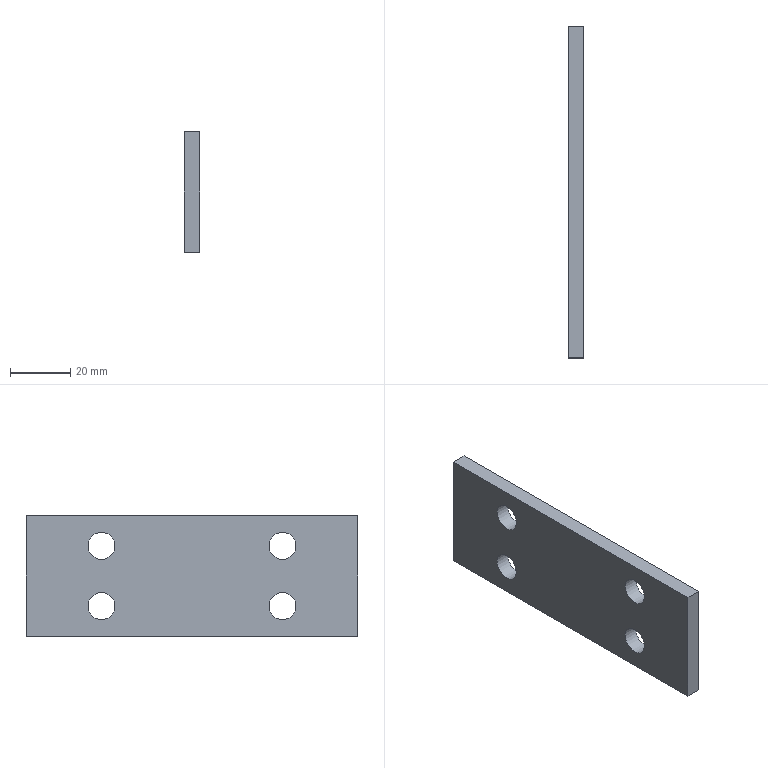Component | NX | CH3404_2-5 | 1 solid | 10 faces | box 5 x 110 x 40 mm | volume 20728 mm3 | plane 6 | cylinder 4 | commonest cylinder face diameters 9 x4
STEP:
#1=CARTESIAN_POINT('',(0.,0.,0.));
#2=DIRECTION('',(0.,0.,1.));
#3=DIRECTION('',(1.,0.,0.));
#4=AXIS2_PLACEMENT_3D('',#1,#2,#3);
#5=CARTESIAN_POINT('',(58.,-55.,20.));
#6=VERTEX_POINT('',#5);
#7=CARTESIAN_POINT('',(58.,-55.,-20.));
#8=VERTEX_POINT('',#7);
#9=CARTESIAN_POINT('',(58.,-55.,20.));
#10=DIRECTION('',(0.,0.,-1.));
#11=VECTOR('',#10,1.);
#12=LINE('',#9,#11);
#13=CARTESIAN_POINT('',(63.,-55.,20.));
#14=DIRECTION('',(0.,1.,0.));
#15=DIRECTION('',(0.,0.,1.));
#16=AXIS2_PLACEMENT_3D('',#13,#14,#15);
#17=PLANE('',#16);
#18=CARTESIAN_POINT('',(0.,-5.));
#19=DIRECTION('',(-1.,0.));
#20=VECTOR('',#19,1.);
#21=LINE('',#18,#20);
#22=(GEOMETRIC_REPRESENTATION_CONTEXT(2)PARAMETRIC_REPRESENTATION_CONTEXT()REPRESENTATION_CONTEXT('',''));
#23=DEFINITIONAL_REPRESENTATION('',(#21),#22);
#24=PCURVE('',#17,#23);
#25=CARTESIAN_POINT('',(58.,-0.,0.));
#26=DIRECTION('',(1.,0.,0.));
#27=DIRECTION('',(0.,0.,-1.));
#28=AXIS2_PLACEMENT_3D('',#25,#26,#27);
#29=PLANE('',#28);
#30=CARTESIAN_POINT('',(-20.,-55.));
#31=DIRECTION('',(1.,0.));
#32=VECTOR('',#31,1.);
#33=LINE('',#30,#32);
#34=(GEOMETRIC_REPRESENTATION_CONTEXT(2)PARAMETRIC_REPRESENTATION_CONTEXT()REPRESENTATION_CONTEXT('',''));
#35=DEFINITIONAL_REPRESENTATION('',(#33),#34);
#36=PCURVE('',#29,#35);
#37=SURFACE_CURVE('',#12,(#24,#36),.PCURVE_S1.);
#38=EDGE_CURVE('',#6,#8,#37,.T.);
#39=ORIENTED_EDGE('',*,*,#38,.T.);
#40=CARTESIAN_POINT('',(63.,-55.,-20.));
#41=VERTEX_POINT('',#40);
#42=CARTESIAN_POINT('',(63.,-55.,-20.));
#43=DIRECTION('',(-1.,0.,0.));
#44=VECTOR('',#43,1.);
#45=LINE('',#42,#44);
#46=CARTESIAN_POINT('',(-40.,0.));
#47=DIRECTION('',(0.,-1.));
#48=VECTOR('',#47,1.);
#49=LINE('',#46,#48);
#50=(GEOMETRIC_REPRESENTATION_CONTEXT(2)PARAMETRIC_REPRESENTATION_CONTEXT()REPRESENTATION_CONTEXT('',''));
#51=DEFINITIONAL_REPRESENTATION('',(#49),#50);
#52=PCURVE('',#17,#51);
#53=CARTESIAN_POINT('',(63.,-55.,-20.));
#54=DIRECTION('',(0.,0.,1.));
#55=DIRECTION('',(1.,0.,0.));
#56=AXIS2_PLACEMENT_3D('',#53,#54,#55);
#57=PLANE('',#56);
#58=CARTESIAN_POINT('',(0.,0.));
#59=DIRECTION('',(-1.,0.));
#60=VECTOR('',#59,1.);
#61=LINE('',#58,#60);
#62=(GEOMETRIC_REPRESENTATION_CONTEXT(2)PARAMETRIC_REPRESENTATION_CONTEXT()REPRESENTATION_CONTEXT('',''));
#63=DEFINITIONAL_REPRESENTATION('',(#61),#62);
#64=PCURVE('',#57,#63);
#65=SURFACE_CURVE('',#45,(#52,#64),.PCURVE_S1.);
#66=EDGE_CURVE('',#41,#8,#65,.T.);
#67=ORIENTED_EDGE('',*,*,#66,.F.);
#68=CARTESIAN_POINT('',(63.,-55.,20.));
#69=VERTEX_POINT('',#68);
#70=CARTESIAN_POINT('',(63.,-55.,20.));
#71=DIRECTION('',(0.,0.,-1.));
#72=VECTOR('',#71,1.);
#73=LINE('',#70,#72);
#74=CARTESIAN_POINT('',(0.,0.));
#75=DIRECTION('',(-1.,0.));
#76=VECTOR('',#75,1.);
#77=LINE('',#74,#76);
#78=(GEOMETRIC_REPRESENTATION_CONTEXT(2)PARAMETRIC_REPRESENTATION_CONTEXT()REPRESENTATION_CONTEXT('',''));
#79=DEFINITIONAL_REPRESENTATION('',(#77),#78);
#80=PCURVE('',#17,#79);
#81=CARTESIAN_POINT('',(63.,-0.,0.));
#82=DIRECTION('',(1.,0.,0.));
#83=DIRECTION('',(0.,0.,-1.));
#84=AXIS2_PLACEMENT_3D('',#81,#82,#83);
#85=PLANE('',#84);
#86=CARTESIAN_POINT('',(-20.,-55.));
#87=DIRECTION('',(1.,0.));
#88=VECTOR('',#87,1.);
#89=LINE('',#86,#88);
#90=(GEOMETRIC_REPRESENTATION_CONTEXT(2)PARAMETRIC_REPRESENTATION_CONTEXT()REPRESENTATION_CONTEXT('',''));
#91=DEFINITIONAL_REPRESENTATION('',(#89),#90);
#92=PCURVE('',#85,#91);
#93=SURFACE_CURVE('',#73,(#80,#92),.PCURVE_S1.);
#94=EDGE_CURVE('',#69,#41,#93,.T.);
#95=ORIENTED_EDGE('',*,*,#94,.F.);
#96=CARTESIAN_POINT('',(63.,-55.,20.));
#97=DIRECTION('',(-1.,0.,0.));
#98=VECTOR('',#97,1.);
#99=LINE('',#96,#98);
#100=CARTESIAN_POINT('',(0.,0.));
#101=DIRECTION('',(0.,-1.));
#102=VECTOR('',#101,1.);
#103=LINE('',#100,#102);
#104=(GEOMETRIC_REPRESENTATION_CONTEXT(2)PARAMETRIC_REPRESENTATION_CONTEXT()REPRESENTATION_CONTEXT('',''));
#105=DEFINITIONAL_REPRESENTATION('',(#103),#104);
#106=PCURVE('',#17,#105);
#107=CARTESIAN_POINT('',(63.,55.,20.));
#108=DIRECTION('',(0.,0.,-1.));
#109=DIRECTION('',(-1.,0.,0.));
#110=AXIS2_PLACEMENT_3D('',#107,#108,#109);
#111=PLANE('',#110);
#112=CARTESIAN_POINT('',(0.,-110.));
#113=DIRECTION('',(1.,0.));
#114=VECTOR('',#113,1.);
#115=LINE('',#112,#114);
#116=(GEOMETRIC_REPRESENTATION_CONTEXT(2)PARAMETRIC_REPRESENTATION_CONTEXT()REPRESENTATION_CONTEXT('',''));
#117=DEFINITIONAL_REPRESENTATION('',(#115),#116);
#118=PCURVE('',#111,#117);
#119=SURFACE_CURVE('',#99,(#106,#118),.PCURVE_S1.);
#120=EDGE_CURVE('',#69,#6,#119,.T.);
#121=ORIENTED_EDGE('',*,*,#120,.T.);
#122=EDGE_LOOP('',(#39,#67,#95,#121));
#123=FACE_BOUND('',#122,.T.);
#124=ADVANCED_FACE('',(#123),#17,.F.);
#125=CARTESIAN_POINT('',(58.,55.,-20.));
#126=VERTEX_POINT('',#125);
#127=CARTESIAN_POINT('',(58.,-55.,-20.));
#128=DIRECTION('',(0.,1.,0.));
#129=VECTOR('',#128,1.);
#130=LINE('',#127,#129);
#131=CARTESIAN_POINT('',(-5.,0.));
#132=DIRECTION('',(0.,1.));
#133=VECTOR('',#132,1.);
#134=LINE('',#131,#133);
#135=(GEOMETRIC_REPRESENTATION_CONTEXT(2)PARAMETRIC_REPRESENTATION_CONTEXT()REPRESENTATION_CONTEXT('',''));
#136=DEFINITIONAL_REPRESENTATION('',(#134),#135);
#137=PCURVE('',#57,#136);
#138=CARTESIAN_POINT('',(20.,-55.));
#139=DIRECTION('',(0.,1.));
#140=VECTOR('',#139,1.);
#141=LINE('',#138,#140);
#142=(GEOMETRIC_REPRESENTATION_CONTEXT(2)PARAMETRIC_REPRESENTATION_CONTEXT()REPRESENTATION_CONTEXT('',''));
#143=DEFINITIONAL_REPRESENTATION('',(#141),#142);
#144=PCURVE('',#29,#143);
#145=SURFACE_CURVE('',#130,(#137,#144),.PCURVE_S1.);
#146=EDGE_CURVE('',#8,#126,#145,.T.);
#147=ORIENTED_EDGE('',*,*,#146,.T.);
#148=CARTESIAN_POINT('',(63.,55.,-20.));
#149=VERTEX_POINT('',#148);
#150=CARTESIAN_POINT('',(63.,55.,-20.));
#151=DIRECTION('',(-1.,0.,0.));
#152=VECTOR('',#151,1.);
#153=LINE('',#150,#152);
#154=CARTESIAN_POINT('',(0.,110.));
#155=DIRECTION('',(-1.,0.));
#156=VECTOR('',#155,1.);
#157=LINE('',#154,#156);
#158=(GEOMETRIC_REPRESENTATION_CONTEXT(2)PARAMETRIC_REPRESENTATION_CONTEXT()REPRESENTATION_CONTEXT('',''));
#159=DEFINITIONAL_REPRESENTATION('',(#157),#158);
#160=PCURVE('',#57,#159);
#161=CARTESIAN_POINT('',(63.,55.,-20.));
#162=DIRECTION('',(0.,-1.,0.));
#163=DIRECTION('',(0.,0.,-1.));
#164=AXIS2_PLACEMENT_3D('',#161,#162,#163);
#165=PLANE('',#164);
#166=CARTESIAN_POINT('',(0.,0.));
#167=DIRECTION('',(0.,-1.));
#168=VECTOR('',#167,1.);
#169=LINE('',#166,#168);
#170=(GEOMETRIC_REPRESENTATION_CONTEXT(2)PARAMETRIC_REPRESENTATION_CONTEXT()REPRESENTATION_CONTEXT('',''));
#171=DEFINITIONAL_REPRESENTATION('',(#169),#170);
#172=PCURVE('',#165,#171);
#173=SURFACE_CURVE('',#153,(#160,#172),.PCURVE_S1.);
#174=EDGE_CURVE('',#149,#126,#173,.T.);
#175=ORIENTED_EDGE('',*,*,#174,.F.);
#176=CARTESIAN_POINT('',(63.,-55.,-20.));
#177=DIRECTION('',(0.,1.,0.));
#178=VECTOR('',#177,1.);
#179=LINE('',#176,#178);
#180=CARTESIAN_POINT('',(0.,0.));
#181=DIRECTION('',(0.,1.));
#182=VECTOR('',#181,1.);
#183=LINE('',#180,#182);
#184=(GEOMETRIC_REPRESENTATION_CONTEXT(2)PARAMETRIC_REPRESENTATION_CONTEXT()REPRESENTATION_CONTEXT('',''));
#185=DEFINITIONAL_REPRESENTATION('',(#183),#184);
#186=PCURVE('',#57,#185);
#187=CARTESIAN_POINT('',(20.,-55.));
#188=DIRECTION('',(0.,1.));
#189=VECTOR('',#188,1.);
#190=LINE('',#187,#189);
#191=(GEOMETRIC_REPRESENTATION_CONTEXT(2)PARAMETRIC_REPRESENTATION_CONTEXT()REPRESENTATION_CONTEXT('',''));
#192=DEFINITIONAL_REPRESENTATION('',(#190),#191);
#193=PCURVE('',#85,#192);
#194=SURFACE_CURVE('',#179,(#186,#193),.PCURVE_S1.);
#195=EDGE_CURVE('',#41,#149,#194,.T.);
#196=ORIENTED_EDGE('',*,*,#195,.F.);
#197=ORIENTED_EDGE('',*,*,#66,.T.);
#198=EDGE_LOOP('',(#147,#175,#196,#197));
#199=FACE_BOUND('',#198,.T.);
#200=ADVANCED_FACE('',(#199),#57,.F.);
#201=CARTESIAN_POINT('',(58.,55.,20.));
#202=VERTEX_POINT('',#201);
#203=CARTESIAN_POINT('',(58.,55.,-20.));
#204=DIRECTION('',(0.,0.,1.));
#205=VECTOR('',#204,1.);
#206=LINE('',#203,#205);
#207=CARTESIAN_POINT('',(0.,-5.));
#208=DIRECTION('',(-1.,0.));
#209=VECTOR('',#208,1.);
#210=LINE('',#207,#209);
#211=(GEOMETRIC_REPRESENTATION_CONTEXT(2)PARAMETRIC_REPRESENTATION_CONTEXT()REPRESENTATION_CONTEXT('',''));
#212=DEFINITIONAL_REPRESENTATION('',(#210),#211);
#213=PCURVE('',#165,#212);
#214=CARTESIAN_POINT('',(20.,55.));
#215=DIRECTION('',(-1.,0.));
#216=VECTOR('',#215,1.);
#217=LINE('',#214,#216);
#218=(GEOMETRIC_REPRESENTATION_CONTEXT(2)PARAMETRIC_REPRESENTATION_CONTEXT()REPRESENTATION_CONTEXT('',''));
#219=DEFINITIONAL_REPRESENTATION('',(#217),#218);
#220=PCURVE('',#29,#219);
#221=SURFACE_CURVE('',#206,(#213,#220),.PCURVE_S1.);
#222=EDGE_CURVE('',#126,#202,#221,.T.);
#223=ORIENTED_EDGE('',*,*,#222,.T.);
#224=CARTESIAN_POINT('',(63.,55.,20.));
#225=VERTEX_POINT('',#224);
#226=CARTESIAN_POINT('',(63.,55.,20.));
#227=DIRECTION('',(-1.,0.,0.));
#228=VECTOR('',#227,1.);
#229=LINE('',#226,#228);
#230=CARTESIAN_POINT('',(-40.,0.));
#231=DIRECTION('',(0.,-1.));
#232=VECTOR('',#231,1.);
#233=LINE('',#230,#232);
#234=(GEOMETRIC_REPRESENTATION_CONTEXT(2)PARAMETRIC_REPRESENTATION_CONTEXT()REPRESENTATION_CONTEXT('',''));
#235=DEFINITIONAL_REPRESENTATION('',(#233),#234);
#236=PCURVE('',#165,#235);
#237=CARTESIAN_POINT('',(0.,0.));
#238=DIRECTION('',(1.,0.));
#239=VECTOR('',#238,1.);
#240=LINE('',#237,#239);
#241=(GEOMETRIC_REPRESENTATION_CONTEXT(2)PARAMETRIC_REPRESENTATION_CONTEXT()REPRESENTATION_CONTEXT('',''));
#242=DEFINITIONAL_REPRESENTATION('',(#240),#241);
#243=PCURVE('',#111,#242);
#244=SURFACE_CURVE('',#229,(#236,#243),.PCURVE_S1.);
#245=EDGE_CURVE('',#225,#202,#244,.T.);
#246=ORIENTED_EDGE('',*,*,#245,.F.);
#247=CARTESIAN_POINT('',(63.,55.,-20.));
#248=DIRECTION('',(0.,0.,1.));
#249=VECTOR('',#248,1.);
#250=LINE('',#247,#249);
#251=CARTESIAN_POINT('',(0.,0.));
#252=DIRECTION('',(-1.,0.));
#253=VECTOR('',#252,1.);
#254=LINE('',#251,#253);
#255=(GEOMETRIC_REPRESENTATION_CONTEXT(2)PARAMETRIC_REPRESENTATION_CONTEXT()REPRESENTATION_CONTEXT('',''));
#256=DEFINITIONAL_REPRESENTATION('',(#254),#255);
#257=PCURVE('',#165,#256);
#258=CARTESIAN_POINT('',(20.,55.));
#259=DIRECTION('',(-1.,0.));
#260=VECTOR('',#259,1.);
#261=LINE('',#258,#260);
#262=(GEOMETRIC_REPRESENTATION_CONTEXT(2)PARAMETRIC_REPRESENTATION_CONTEXT()REPRESENTATION_CONTEXT('',''));
#263=DEFINITIONAL_REPRESENTATION('',(#261),#262);
#264=PCURVE('',#85,#263);
#265=SURFACE_CURVE('',#250,(#257,#264),.PCURVE_S1.);
#266=EDGE_CURVE('',#149,#225,#265,.T.);
#267=ORIENTED_EDGE('',*,*,#266,.F.);
#268=ORIENTED_EDGE('',*,*,#174,.T.);
#269=EDGE_LOOP('',(#223,#246,#267,#268));
#270=FACE_BOUND('',#269,.T.);
#271=ADVANCED_FACE('',(#270),#165,.F.);
#272=CARTESIAN_POINT('',(58.,55.,20.));
#273=DIRECTION('',(0.,-1.,0.));
#274=VECTOR('',#273,1.);
#275=LINE('',#272,#274);
#276=CARTESIAN_POINT('',(5.,0.));
#277=DIRECTION('',(0.,-1.));
#278=VECTOR('',#277,1.);
#279=LINE('',#276,#278);
#280=(GEOMETRIC_REPRESENTATION_CONTEXT(2)PARAMETRIC_REPRESENTATION_CONTEXT()REPRESENTATION_CONTEXT('',''));
#281=DEFINITIONAL_REPRESENTATION('',(#279),#280);
#282=PCURVE('',#111,#281);
#283=CARTESIAN_POINT('',(-20.,55.));
#284=DIRECTION('',(0.,-1.));
#285=VECTOR('',#284,1.);
#286=LINE('',#283,#285);
#287=(GEOMETRIC_REPRESENTATION_CONTEXT(2)PARAMETRIC_REPRESENTATION_CONTEXT()REPRESENTATION_CONTEXT('',''));
#288=DEFINITIONAL_REPRESENTATION('',(#286),#287);
#289=PCURVE('',#29,#288);
#290=SURFACE_CURVE('',#275,(#282,#289),.PCURVE_S1.);
#291=EDGE_CURVE('',#202,#6,#290,.T.);
#292=ORIENTED_EDGE('',*,*,#291,.T.);
#293=ORIENTED_EDGE('',*,*,#120,.F.);
#294=CARTESIAN_POINT('',(63.,55.,20.));
#295=DIRECTION('',(0.,-1.,0.));
#296=VECTOR('',#295,1.);
#297=LINE('',#294,#296);
#298=CARTESIAN_POINT('',(0.,0.));
#299=DIRECTION('',(0.,-1.));
#300=VECTOR('',#299,1.);
#301=LINE('',#298,#300);
#302=(GEOMETRIC_REPRESENTATION_CONTEXT(2)PARAMETRIC_REPRESENTATION_CONTEXT()REPRESENTATION_CONTEXT('',''));
#303=DEFINITIONAL_REPRESENTATION('',(#301),#302);
#304=PCURVE('',#111,#303);
#305=CARTESIAN_POINT('',(-20.,55.));
#306=DIRECTION('',(0.,-1.));
#307=VECTOR('',#306,1.);
#308=LINE('',#305,#307);
#309=(GEOMETRIC_REPRESENTATION_CONTEXT(2)PARAMETRIC_REPRESENTATION_CONTEXT()REPRESENTATION_CONTEXT('',''));
#310=DEFINITIONAL_REPRESENTATION('',(#308),#309);
#311=PCURVE('',#85,#310);
#312=SURFACE_CURVE('',#297,(#304,#311),.PCURVE_S1.);
#313=EDGE_CURVE('',#225,#69,#312,.T.);
#314=ORIENTED_EDGE('',*,*,#313,.F.);
#315=ORIENTED_EDGE('',*,*,#245,.T.);
#316=EDGE_LOOP('',(#292,#293,#314,#315));
#317=FACE_BOUND('',#316,.T.);
#318=ADVANCED_FACE('',(#317),#111,.F.);
#319=CARTESIAN_POINT('',(63.,30.,14.5));
#320=VERTEX_POINT('',#319);
#321=CARTESIAN_POINT('',(63.,30.,10.));
#322=DIRECTION('',(-1.,0.,0.));
#323=DIRECTION('',(0.,0.,1.));
#324=AXIS2_PLACEMENT_3D('',#321,#322,#323);
#325=CIRCLE('',#324,4.5);
#326=CARTESIAN_POINT('',(-14.5,30.));
#327=CARTESIAN_POINT('',(-14.5,37.794));
#328=CARTESIAN_POINT('',(-7.75,33.897));
#329=CARTESIAN_POINT('',(-1.,30.));
#330=CARTESIAN_POINT('',(-7.75,26.103));
#331=CARTESIAN_POINT('',(-14.5,22.206));
#332=CARTESIAN_POINT('',(-14.5,30.));
#333=(BOUNDED_CURVE()B_SPLINE_CURVE(2,(#326,#327,#328,#329,#330,#331,#332),.UNSPECIFIED.,.T.,.F.)B_SPLINE_CURVE_WITH_KNOTS((1,2,2,2,2,1),(-2.094,0.,2.094,4.189,6.283,8.378),.UNSPECIFIED.)CURVE()GEOMETRIC_REPRESENTATION_ITEM()RATIONAL_B_SPLINE_CURVE((1.,0.5,1.,0.5,1.,0.5,1.))REPRESENTATION_ITEM(''));
#334=(GEOMETRIC_REPRESENTATION_CONTEXT(2)PARAMETRIC_REPRESENTATION_CONTEXT()REPRESENTATION_CONTEXT('',''));
#335=DEFINITIONAL_REPRESENTATION('',(#333),#334);
#336=PCURVE('',#85,#335);
#337=CARTESIAN_POINT('',(63.,30.,10.));
#338=DIRECTION('',(-1.,0.,0.));
#339=DIRECTION('',(0.,0.,1.));
#340=AXIS2_PLACEMENT_3D('',#337,#338,#339);
#341=CYLINDRICAL_SURFACE('',#340,4.5);
#342=CARTESIAN_POINT('',(0.,0.));
#343=DIRECTION('',(1.,0.));
#344=VECTOR('',#343,1.);
#345=LINE('',#342,#344);
#346=(GEOMETRIC_REPRESENTATION_CONTEXT(2)PARAMETRIC_REPRESENTATION_CONTEXT()REPRESENTATION_CONTEXT('',''));
#347=DEFINITIONAL_REPRESENTATION('',(#345),#346);
#348=PCURVE('',#341,#347);
#349=SURFACE_CURVE('',#325,(#336,#348),.PCURVE_S1.);
#350=EDGE_CURVE('',#320,#320,#349,.T.);
#351=ORIENTED_EDGE('',*,*,#350,.T.);
#352=EDGE_LOOP('',(#351));
#353=FACE_BOUND('',#352,.T.);
#354=CARTESIAN_POINT('',(63.,30.,-5.5));
#355=VERTEX_POINT('',#354);
#356=CARTESIAN_POINT('',(63.,30.,-10.));
#357=DIRECTION('',(-1.,0.,0.));
#358=DIRECTION('',(0.,0.,1.));
#359=AXIS2_PLACEMENT_3D('',#356,#357,#358);
#360=CIRCLE('',#359,4.5);
#361=CARTESIAN_POINT('',(5.5,30.));
#362=CARTESIAN_POINT('',(5.5,37.794));
#363=CARTESIAN_POINT('',(12.25,33.897));
#364=CARTESIAN_POINT('',(19.,30.));
#365=CARTESIAN_POINT('',(12.25,26.103));
#366=CARTESIAN_POINT('',(5.5,22.206));
#367=CARTESIAN_POINT('',(5.5,30.));
#368=(BOUNDED_CURVE()B_SPLINE_CURVE(2,(#361,#362,#363,#364,#365,#366,#367),.UNSPECIFIED.,.T.,.F.)B_SPLINE_CURVE_WITH_KNOTS((1,2,2,2,2,1),(-2.094,0.,2.094,4.189,6.283,8.378),.UNSPECIFIED.)CURVE()GEOMETRIC_REPRESENTATION_ITEM()RATIONAL_B_SPLINE_CURVE((1.,0.5,1.,0.5,1.,0.5,1.))REPRESENTATION_ITEM(''));
#369=(GEOMETRIC_REPRESENTATION_CONTEXT(2)PARAMETRIC_REPRESENTATION_CONTEXT()REPRESENTATION_CONTEXT('',''));
#370=DEFINITIONAL_REPRESENTATION('',(#368),#369);
#371=PCURVE('',#85,#370);
#372=CARTESIAN_POINT('',(63.,30.,-10.));
#373=DIRECTION('',(-1.,0.,0.));
#374=DIRECTION('',(0.,0.,1.));
#375=AXIS2_PLACEMENT_3D('',#372,#373,#374);
#376=CYLINDRICAL_SURFACE('',#375,4.5);
#377=CARTESIAN_POINT('',(0.,0.));
#378=DIRECTION('',(1.,0.));
#379=VECTOR('',#378,1.);
#380=LINE('',#377,#379);
#381=(GEOMETRIC_REPRESENTATION_CONTEXT(2)PARAMETRIC_REPRESENTATION_CONTEXT()REPRESENTATION_CONTEXT('',''));
#382=DEFINITIONAL_REPRESENTATION('',(#380),#381);
#383=PCURVE('',#376,#382);
#384=SURFACE_CURVE('',#360,(#371,#383),.PCURVE_S1.);
#385=EDGE_CURVE('',#355,#355,#384,.T.);
#386=ORIENTED_EDGE('',*,*,#385,.T.);
#387=EDGE_LOOP('',(#386));
#388=FACE_BOUND('',#387,.T.);
#389=CARTESIAN_POINT('',(63.,-30.,14.5));
#390=VERTEX_POINT('',#389);
#391=CARTESIAN_POINT('',(63.,-30.,10.));
#392=DIRECTION('',(-1.,0.,0.));
#393=DIRECTION('',(0.,0.,1.));
#394=AXIS2_PLACEMENT_3D('',#391,#392,#393);
#395=CIRCLE('',#394,4.5);
#396=CARTESIAN_POINT('',(-14.5,-30.));
#397=CARTESIAN_POINT('',(-14.5,-22.206));
#398=CARTESIAN_POINT('',(-7.75,-26.103));
#399=CARTESIAN_POINT('',(-1.,-30.));
#400=CARTESIAN_POINT('',(-7.75,-33.897));
#401=CARTESIAN_POINT('',(-14.5,-37.794));
#402=CARTESIAN_POINT('',(-14.5,-30.));
#403=(BOUNDED_CURVE()B_SPLINE_CURVE(2,(#396,#397,#398,#399,#400,#401,#402),.UNSPECIFIED.,.T.,.F.)B_SPLINE_CURVE_WITH_KNOTS((1,2,2,2,2,1),(-2.094,0.,2.094,4.189,6.283,8.378),.UNSPECIFIED.)CURVE()GEOMETRIC_REPRESENTATION_ITEM()RATIONAL_B_SPLINE_CURVE((1.,0.5,1.,0.5,1.,0.5,1.))REPRESENTATION_ITEM(''));
#404=(GEOMETRIC_REPRESENTATION_CONTEXT(2)PARAMETRIC_REPRESENTATION_CONTEXT()REPRESENTATION_CONTEXT('',''));
#405=DEFINITIONAL_REPRESENTATION('',(#403),#404);
#406=PCURVE('',#85,#405);
#407=CARTESIAN_POINT('',(63.,-30.,10.));
#408=DIRECTION('',(-1.,0.,0.));
#409=DIRECTION('',(0.,0.,1.));
#410=AXIS2_PLACEMENT_3D('',#407,#408,#409);
#411=CYLINDRICAL_SURFACE('',#410,4.5);
#412=CARTESIAN_POINT('',(0.,0.));
#413=DIRECTION('',(1.,0.));
#414=VECTOR('',#413,1.);
#415=LINE('',#412,#414);
#416=(GEOMETRIC_REPRESENTATION_CONTEXT(2)PARAMETRIC_REPRESENTATION_CONTEXT()REPRESENTATION_CONTEXT('',''));
#417=DEFINITIONAL_REPRESENTATION('',(#415),#416);
#418=PCURVE('',#411,#417);
#419=SURFACE_CURVE('',#395,(#406,#418),.PCURVE_S1.);
#420=EDGE_CURVE('',#390,#390,#419,.T.);
#421=ORIENTED_EDGE('',*,*,#420,.T.);
#422=EDGE_LOOP('',(#421));
#423=FACE_BOUND('',#422,.T.);
#424=CARTESIAN_POINT('',(63.,-30.,-5.5));
#425=VERTEX_POINT('',#424);
#426=CARTESIAN_POINT('',(63.,-30.,-10.));
#427=DIRECTION('',(-1.,0.,0.));
#428=DIRECTION('',(0.,0.,1.));
#429=AXIS2_PLACEMENT_3D('',#426,#427,#428);
#430=CIRCLE('',#429,4.5);
#431=CARTESIAN_POINT('',(5.5,-30.));
#432=CARTESIAN_POINT('',(5.5,-22.206));
#433=CARTESIAN_POINT('',(12.25,-26.103));
#434=CARTESIAN_POINT('',(19.,-30.));
#435=CARTESIAN_POINT('',(12.25,-33.897));
#436=CARTESIAN_POINT('',(5.5,-37.794));
#437=CARTESIAN_POINT('',(5.5,-30.));
#438=(BOUNDED_CURVE()B_SPLINE_CURVE(2,(#431,#432,#433,#434,#435,#436,#437),.UNSPECIFIED.,.T.,.F.)B_SPLINE_CURVE_WITH_KNOTS((1,2,2,2,2,1),(-2.094,0.,2.094,4.189,6.283,8.378),.UNSPECIFIED.)CURVE()GEOMETRIC_REPRESENTATION_ITEM()RATIONAL_B_SPLINE_CURVE((1.,0.5,1.,0.5,1.,0.5,1.))REPRESENTATION_ITEM(''));
#439=(GEOMETRIC_REPRESENTATION_CONTEXT(2)PARAMETRIC_REPRESENTATION_CONTEXT()REPRESENTATION_CONTEXT('',''));
#440=DEFINITIONAL_REPRESENTATION('',(#438),#439);
#441=PCURVE('',#85,#440);
#442=CARTESIAN_POINT('',(63.,-30.,-10.));
#443=DIRECTION('',(-1.,0.,0.));
#444=DIRECTION('',(0.,0.,1.));
#445=AXIS2_PLACEMENT_3D('',#442,#443,#444);
#446=CYLINDRICAL_SURFACE('',#445,4.5);
#447=CARTESIAN_POINT('',(0.,0.));
#448=DIRECTION('',(1.,0.));
#449=VECTOR('',#448,1.);
#450=LINE('',#447,#449);
#451=(GEOMETRIC_REPRESENTATION_CONTEXT(2)PARAMETRIC_REPRESENTATION_CONTEXT()REPRESENTATION_CONTEXT('',''));
#452=DEFINITIONAL_REPRESENTATION('',(#450),#451);
#453=PCURVE('',#446,#452);
#454=SURFACE_CURVE('',#430,(#441,#453),.PCURVE_S1.);
#455=EDGE_CURVE('',#425,#425,#454,.T.);
#456=ORIENTED_EDGE('',*,*,#455,.T.);
#457=EDGE_LOOP('',(#456));
#458=FACE_BOUND('',#457,.T.);
#459=ORIENTED_EDGE('',*,*,#94,.T.);
#460=ORIENTED_EDGE('',*,*,#195,.T.);
#461=ORIENTED_EDGE('',*,*,#266,.T.);
#462=ORIENTED_EDGE('',*,*,#313,.T.);
#463=EDGE_LOOP('',(#459,#460,#461,#462));
#464=FACE_BOUND('',#463,.T.);
#465=ADVANCED_FACE('',(#353,#388,#423,#458,#464),#85,.T.);
#466=CARTESIAN_POINT('',(58.,30.,5.5));
#467=VERTEX_POINT('',#466);
#468=CARTESIAN_POINT('',(58.,30.,14.5));
#469=VERTEX_POINT('',#468);
#470=CARTESIAN_POINT('',(58.,30.,10.));
#471=DIRECTION('',(1.,0.,0.));
#472=DIRECTION('',(0.,0.,-1.));
#473=AXIS2_PLACEMENT_3D('',#470,#471,#472);
#474=CIRCLE('',#473,4.5);
#475=CARTESIAN_POINT('',(-10.,30.));
#476=DIRECTION('',(1.,0.));
#477=AXIS2_PLACEMENT_2D('',#475,#476);
#478=CIRCLE('',#477,4.5);
#479=(GEOMETRIC_REPRESENTATION_CONTEXT(2)PARAMETRIC_REPRESENTATION_CONTEXT()REPRESENTATION_CONTEXT('',''));
#480=DEFINITIONAL_REPRESENTATION('',(#478),#479);
#481=PCURVE('',#29,#480);
#482=CARTESIAN_POINT('',(3.142,5.));
#483=DIRECTION('',(-1.,0.));
#484=VECTOR('',#483,1.);
#485=LINE('',#482,#484);
#486=(GEOMETRIC_REPRESENTATION_CONTEXT(2)PARAMETRIC_REPRESENTATION_CONTEXT()REPRESENTATION_CONTEXT('',''));
#487=DEFINITIONAL_REPRESENTATION('',(#485),#486);
#488=PCURVE('',#341,#487);
#489=SURFACE_CURVE('',#474,(#481,#488),.PCURVE_S1.);
#490=EDGE_CURVE('',#467,#469,#489,.T.);
#491=ORIENTED_EDGE('',*,*,#490,.T.);
#492=CARTESIAN_POINT('',(58.,30.,10.));
#493=DIRECTION('',(1.,0.,0.));
#494=DIRECTION('',(0.,0.,-1.));
#495=AXIS2_PLACEMENT_3D('',#492,#493,#494);
#496=CIRCLE('',#495,4.5);
#497=CARTESIAN_POINT('',(-10.,30.));
#498=DIRECTION('',(1.,0.));
#499=AXIS2_PLACEMENT_2D('',#497,#498);
#500=CIRCLE('',#499,4.5);
#501=(GEOMETRIC_REPRESENTATION_CONTEXT(2)PARAMETRIC_REPRESENTATION_CONTEXT()REPRESENTATION_CONTEXT('',''));
#502=DEFINITIONAL_REPRESENTATION('',(#500),#501);
#503=PCURVE('',#29,#502);
#504=CARTESIAN_POINT('',(9.425,5.));
#505=DIRECTION('',(-1.,0.));
#506=VECTOR('',#505,1.);
#507=LINE('',#504,#506);
#508=(GEOMETRIC_REPRESENTATION_CONTEXT(2)PARAMETRIC_REPRESENTATION_CONTEXT()REPRESENTATION_CONTEXT('',''));
#509=DEFINITIONAL_REPRESENTATION('',(#507),#508);
#510=PCURVE('',#341,#509);
#511=SURFACE_CURVE('',#496,(#503,#510),.PCURVE_S1.);
#512=EDGE_CURVE('',#469,#467,#511,.T.);
#513=ORIENTED_EDGE('',*,*,#512,.T.);
#514=EDGE_LOOP('',(#491,#513));
#515=FACE_BOUND('',#514,.T.);
#516=CARTESIAN_POINT('',(58.,30.,-14.5));
#517=VERTEX_POINT('',#516);
#518=CARTESIAN_POINT('',(58.,30.,-5.5));
#519=VERTEX_POINT('',#518);
#520=CARTESIAN_POINT('',(58.,30.,-10.));
#521=DIRECTION('',(1.,0.,0.));
#522=DIRECTION('',(0.,0.,-1.));
#523=AXIS2_PLACEMENT_3D('',#520,#521,#522);
#524=CIRCLE('',#523,4.5);
#525=CARTESIAN_POINT('',(10.,30.));
#526=DIRECTION('',(1.,0.));
#527=AXIS2_PLACEMENT_2D('',#525,#526);
#528=CIRCLE('',#527,4.5);
#529=(GEOMETRIC_REPRESENTATION_CONTEXT(2)PARAMETRIC_REPRESENTATION_CONTEXT()REPRESENTATION_CONTEXT('',''));
#530=DEFINITIONAL_REPRESENTATION('',(#528),#529);
#531=PCURVE('',#29,#530);
#532=CARTESIAN_POINT('',(3.142,5.));
#533=DIRECTION('',(-1.,0.));
#534=VECTOR('',#533,1.);
#535=LINE('',#532,#534);
#536=(GEOMETRIC_REPRESENTATION_CONTEXT(2)PARAMETRIC_REPRESENTATION_CONTEXT()REPRESENTATION_CONTEXT('',''));
#537=DEFINITIONAL_REPRESENTATION('',(#535),#536);
#538=PCURVE('',#376,#537);
#539=SURFACE_CURVE('',#524,(#531,#538),.PCURVE_S1.);
#540=EDGE_CURVE('',#517,#519,#539,.T.);
#541=ORIENTED_EDGE('',*,*,#540,.T.);
#542=CARTESIAN_POINT('',(58.,30.,-10.));
#543=DIRECTION('',(1.,0.,0.));
#544=DIRECTION('',(0.,0.,-1.));
#545=AXIS2_PLACEMENT_3D('',#542,#543,#544);
#546=CIRCLE('',#545,4.5);
#547=CARTESIAN_POINT('',(10.,30.));
#548=DIRECTION('',(1.,0.));
#549=AXIS2_PLACEMENT_2D('',#547,#548);
#550=CIRCLE('',#549,4.5);
#551=(GEOMETRIC_REPRESENTATION_CONTEXT(2)PARAMETRIC_REPRESENTATION_CONTEXT()REPRESENTATION_CONTEXT('',''));
#552=DEFINITIONAL_REPRESENTATION('',(#550),#551);
#553=PCURVE('',#29,#552);
#554=CARTESIAN_POINT('',(9.425,5.));
#555=DIRECTION('',(-1.,0.));
#556=VECTOR('',#555,1.);
#557=LINE('',#554,#556);
#558=(GEOMETRIC_REPRESENTATION_CONTEXT(2)PARAMETRIC_REPRESENTATION_CONTEXT()REPRESENTATION_CONTEXT('',''));
#559=DEFINITIONAL_REPRESENTATION('',(#557),#558);
#560=PCURVE('',#376,#559);
#561=SURFACE_CURVE('',#546,(#553,#560),.PCURVE_S1.);
#562=EDGE_CURVE('',#519,#517,#561,.T.);
#563=ORIENTED_EDGE('',*,*,#562,.T.);
#564=EDGE_LOOP('',(#541,#563));
#565=FACE_BOUND('',#564,.T.);
#566=CARTESIAN_POINT('',(58.,-30.,5.5));
#567=VERTEX_POINT('',#566);
#568=CARTESIAN_POINT('',(58.,-30.,14.5));
#569=VERTEX_POINT('',#568);
#570=CARTESIAN_POINT('',(58.,-30.,10.));
#571=DIRECTION('',(1.,0.,0.));
#572=DIRECTION('',(0.,0.,-1.));
#573=AXIS2_PLACEMENT_3D('',#570,#571,#572);
#574=CIRCLE('',#573,4.5);
#575=CARTESIAN_POINT('',(-10.,-30.));
#576=DIRECTION('',(1.,0.));
#577=AXIS2_PLACEMENT_2D('',#575,#576);
#578=CIRCLE('',#577,4.5);
#579=(GEOMETRIC_REPRESENTATION_CONTEXT(2)PARAMETRIC_REPRESENTATION_CONTEXT()REPRESENTATION_CONTEXT('',''));
#580=DEFINITIONAL_REPRESENTATION('',(#578),#579);
#581=PCURVE('',#29,#580);
#582=CARTESIAN_POINT('',(3.142,5.));
#583=DIRECTION('',(-1.,0.));
#584=VECTOR('',#583,1.);
#585=LINE('',#582,#584);
#586=(GEOMETRIC_REPRESENTATION_CONTEXT(2)PARAMETRIC_REPRESENTATION_CONTEXT()REPRESENTATION_CONTEXT('',''));
#587=DEFINITIONAL_REPRESENTATION('',(#585),#586);
#588=PCURVE('',#411,#587);
#589=SURFACE_CURVE('',#574,(#581,#588),.PCURVE_S1.);
#590=EDGE_CURVE('',#567,#569,#589,.T.);
#591=ORIENTED_EDGE('',*,*,#590,.T.);
#592=CARTESIAN_POINT('',(58.,-30.,10.));
#593=DIRECTION('',(1.,0.,0.));
#594=DIRECTION('',(0.,0.,-1.));
#595=AXIS2_PLACEMENT_3D('',#592,#593,#594);
#596=CIRCLE('',#595,4.5);
#597=CARTESIAN_POINT('',(-10.,-30.));
#598=DIRECTION('',(1.,0.));
#599=AXIS2_PLACEMENT_2D('',#597,#598);
#600=CIRCLE('',#599,4.5);
#601=(GEOMETRIC_REPRESENTATION_CONTEXT(2)PARAMETRIC_REPRESENTATION_CONTEXT()REPRESENTATION_CONTEXT('',''));
#602=DEFINITIONAL_REPRESENTATION('',(#600),#601);
#603=PCURVE('',#29,#602);
#604=CARTESIAN_POINT('',(9.425,5.));
#605=DIRECTION('',(-1.,0.));
#606=VECTOR('',#605,1.);
#607=LINE('',#604,#606);
#608=(GEOMETRIC_REPRESENTATION_CONTEXT(2)PARAMETRIC_REPRESENTATION_CONTEXT()REPRESENTATION_CONTEXT('',''));
#609=DEFINITIONAL_REPRESENTATION('',(#607),#608);
#610=PCURVE('',#411,#609);
#611=SURFACE_CURVE('',#596,(#603,#610),.PCURVE_S1.);
#612=EDGE_CURVE('',#569,#567,#611,.T.);
#613=ORIENTED_EDGE('',*,*,#612,.T.);
#614=EDGE_LOOP('',(#591,#613));
#615=FACE_BOUND('',#614,.T.);
#616=CARTESIAN_POINT('',(58.,-30.,-14.5));
#617=VERTEX_POINT('',#616);
#618=CARTESIAN_POINT('',(58.,-30.,-5.5));
#619=VERTEX_POINT('',#618);
#620=CARTESIAN_POINT('',(58.,-30.,-10.));
#621=DIRECTION('',(1.,0.,0.));
#622=DIRECTION('',(0.,0.,-1.));
#623=AXIS2_PLACEMENT_3D('',#620,#621,#622);
#624=CIRCLE('',#623,4.5);
#625=CARTESIAN_POINT('',(10.,-30.));
#626=DIRECTION('',(1.,0.));
#627=AXIS2_PLACEMENT_2D('',#625,#626);
#628=CIRCLE('',#627,4.5);
#629=(GEOMETRIC_REPRESENTATION_CONTEXT(2)PARAMETRIC_REPRESENTATION_CONTEXT()REPRESENTATION_CONTEXT('',''));
#630=DEFINITIONAL_REPRESENTATION('',(#628),#629);
#631=PCURVE('',#29,#630);
#632=CARTESIAN_POINT('',(3.142,5.));
#633=DIRECTION('',(-1.,0.));
#634=VECTOR('',#633,1.);
#635=LINE('',#632,#634);
#636=(GEOMETRIC_REPRESENTATION_CONTEXT(2)PARAMETRIC_REPRESENTATION_CONTEXT()REPRESENTATION_CONTEXT('',''));
#637=DEFINITIONAL_REPRESENTATION('',(#635),#636);
#638=PCURVE('',#446,#637);
#639=SURFACE_CURVE('',#624,(#631,#638),.PCURVE_S1.);
#640=EDGE_CURVE('',#617,#619,#639,.T.);
#641=ORIENTED_EDGE('',*,*,#640,.T.);
#642=CARTESIAN_POINT('',(58.,-30.,-10.));
#643=DIRECTION('',(1.,0.,0.));
#644=DIRECTION('',(0.,0.,-1.));
#645=AXIS2_PLACEMENT_3D('',#642,#643,#644);
#646=CIRCLE('',#645,4.5);
#647=CARTESIAN_POINT('',(10.,-30.));
#648=DIRECTION('',(1.,0.));
#649=AXIS2_PLACEMENT_2D('',#647,#648);
#650=CIRCLE('',#649,4.5);
#651=(GEOMETRIC_REPRESENTATION_CONTEXT(2)PARAMETRIC_REPRESENTATION_CONTEXT()REPRESENTATION_CONTEXT('',''));
#652=DEFINITIONAL_REPRESENTATION('',(#650),#651);
#653=PCURVE('',#29,#652);
#654=CARTESIAN_POINT('',(9.425,5.));
#655=DIRECTION('',(-1.,0.));
#656=VECTOR('',#655,1.);
#657=LINE('',#654,#656);
#658=(GEOMETRIC_REPRESENTATION_CONTEXT(2)PARAMETRIC_REPRESENTATION_CONTEXT()REPRESENTATION_CONTEXT('',''));
#659=DEFINITIONAL_REPRESENTATION('',(#657),#658);
#660=PCURVE('',#446,#659);
#661=SURFACE_CURVE('',#646,(#653,#660),.PCURVE_S1.);
#662=EDGE_CURVE('',#619,#617,#661,.T.);
#663=ORIENTED_EDGE('',*,*,#662,.T.);
#664=EDGE_LOOP('',(#641,#663));
#665=FACE_BOUND('',#664,.T.);
#666=ORIENTED_EDGE('',*,*,#38,.F.);
#667=ORIENTED_EDGE('',*,*,#291,.F.);
#668=ORIENTED_EDGE('',*,*,#222,.F.);
#669=ORIENTED_EDGE('',*,*,#146,.F.);
#670=EDGE_LOOP('',(#666,#667,#668,#669));
#671=FACE_BOUND('',#670,.T.);
#672=ADVANCED_FACE('',(#515,#565,#615,#665,#671),#29,.F.);
#673=ORIENTED_EDGE('',*,*,#455,.T.);
#674=CARTESIAN_POINT('',(63.,-30.,-5.5));
#675=CARTESIAN_POINT('',(58.,-30.,-5.5));
#676=B_SPLINE_CURVE_WITH_KNOTS('',1,(#674,#675),.UNSPECIFIED.,.F.,.F.,(2,2),(0.,5.),.PIECEWISE_BEZIER_KNOTS.);
#677=CARTESIAN_POINT('',(6.283,0.));
#678=DIRECTION('',(0.,1.));
#679=VECTOR('',#678,1.);
#680=LINE('',#677,#679);
#681=(GEOMETRIC_REPRESENTATION_CONTEXT(2)PARAMETRIC_REPRESENTATION_CONTEXT()REPRESENTATION_CONTEXT('',''));
#682=DEFINITIONAL_REPRESENTATION('',(#680),#681);
#683=PCURVE('',#446,#682);
#684=CARTESIAN_POINT('',(0.,0.));
#685=DIRECTION('',(0.,1.));
#686=VECTOR('',#685,1.);
#687=LINE('',#684,#686);
#688=(GEOMETRIC_REPRESENTATION_CONTEXT(2)PARAMETRIC_REPRESENTATION_CONTEXT()REPRESENTATION_CONTEXT('',''));
#689=DEFINITIONAL_REPRESENTATION('',(#687),#688);
#690=PCURVE('',#446,#689);
#691=SEAM_CURVE('',#676,(#683,#690),.PCURVE_S1.);
#692=EDGE_CURVE('',#425,#619,#691,.T.);
#693=ORIENTED_EDGE('',*,*,#692,.T.);
#694=ORIENTED_EDGE('',*,*,#662,.T.);
#695=ORIENTED_EDGE('',*,*,#640,.T.);
#696=ORIENTED_EDGE('',*,*,#692,.F.);
#697=EDGE_LOOP('',(#673,#693,#694,#695,#696));
#698=FACE_BOUND('',#697,.F.);
#699=ADVANCED_FACE('',(#698),#446,.F.);
#700=ORIENTED_EDGE('',*,*,#420,.T.);
#701=CARTESIAN_POINT('',(63.,-30.,14.5));
#702=CARTESIAN_POINT('',(58.,-30.,14.5));
#703=B_SPLINE_CURVE_WITH_KNOTS('',1,(#701,#702),.UNSPECIFIED.,.F.,.F.,(2,2),(0.,5.),.PIECEWISE_BEZIER_KNOTS.);
#704=CARTESIAN_POINT('',(6.283,0.));
#705=DIRECTION('',(0.,1.));
#706=VECTOR('',#705,1.);
#707=LINE('',#704,#706);
#708=(GEOMETRIC_REPRESENTATION_CONTEXT(2)PARAMETRIC_REPRESENTATION_CONTEXT()REPRESENTATION_CONTEXT('',''));
#709=DEFINITIONAL_REPRESENTATION('',(#707),#708);
#710=PCURVE('',#411,#709);
#711=CARTESIAN_POINT('',(0.,0.));
#712=DIRECTION('',(0.,1.));
#713=VECTOR('',#712,1.);
#714=LINE('',#711,#713);
#715=(GEOMETRIC_REPRESENTATION_CONTEXT(2)PARAMETRIC_REPRESENTATION_CONTEXT()REPRESENTATION_CONTEXT('',''));
#716=DEFINITIONAL_REPRESENTATION('',(#714),#715);
#717=PCURVE('',#411,#716);
#718=SEAM_CURVE('',#703,(#710,#717),.PCURVE_S1.);
#719=EDGE_CURVE('',#390,#569,#718,.T.);
#720=ORIENTED_EDGE('',*,*,#719,.T.);
#721=ORIENTED_EDGE('',*,*,#612,.T.);
#722=ORIENTED_EDGE('',*,*,#590,.T.);
#723=ORIENTED_EDGE('',*,*,#719,.F.);
#724=EDGE_LOOP('',(#700,#720,#721,#722,#723));
#725=FACE_BOUND('',#724,.F.);
#726=ADVANCED_FACE('',(#725),#411,.F.);
#727=ORIENTED_EDGE('',*,*,#385,.T.);
#728=CARTESIAN_POINT('',(63.,30.,-5.5));
#729=CARTESIAN_POINT('',(58.,30.,-5.5));
#730=B_SPLINE_CURVE_WITH_KNOTS('',1,(#728,#729),.UNSPECIFIED.,.F.,.F.,(2,2),(0.,5.),.PIECEWISE_BEZIER_KNOTS.);
#731=CARTESIAN_POINT('',(6.283,0.));
#732=DIRECTION('',(0.,1.));
#733=VECTOR('',#732,1.);
#734=LINE('',#731,#733);
#735=(GEOMETRIC_REPRESENTATION_CONTEXT(2)PARAMETRIC_REPRESENTATION_CONTEXT()REPRESENTATION_CONTEXT('',''));
#736=DEFINITIONAL_REPRESENTATION('',(#734),#735);
#737=PCURVE('',#376,#736);
#738=CARTESIAN_POINT('',(0.,0.));
#739=DIRECTION('',(0.,1.));
#740=VECTOR('',#739,1.);
#741=LINE('',#738,#740);
#742=(GEOMETRIC_REPRESENTATION_CONTEXT(2)PARAMETRIC_REPRESENTATION_CONTEXT()REPRESENTATION_CONTEXT('',''));
#743=DEFINITIONAL_REPRESENTATION('',(#741),#742);
#744=PCURVE('',#376,#743);
#745=SEAM_CURVE('',#730,(#737,#744),.PCURVE_S1.);
#746=EDGE_CURVE('',#355,#519,#745,.T.);
#747=ORIENTED_EDGE('',*,*,#746,.T.);
#748=ORIENTED_EDGE('',*,*,#562,.T.);
#749=ORIENTED_EDGE('',*,*,#540,.T.);
#750=ORIENTED_EDGE('',*,*,#746,.F.);
#751=EDGE_LOOP('',(#727,#747,#748,#749,#750));
#752=FACE_BOUND('',#751,.F.);
#753=ADVANCED_FACE('',(#752),#376,.F.);
#754=ORIENTED_EDGE('',*,*,#350,.T.);
#755=CARTESIAN_POINT('',(63.,30.,14.5));
#756=CARTESIAN_POINT('',(58.,30.,14.5));
#757=B_SPLINE_CURVE_WITH_KNOTS('',1,(#755,#756),.UNSPECIFIED.,.F.,.F.,(2,2),(0.,5.),.PIECEWISE_BEZIER_KNOTS.);
#758=CARTESIAN_POINT('',(6.283,0.));
#759=DIRECTION('',(0.,1.));
#760=VECTOR('',#759,1.);
#761=LINE('',#758,#760);
#762=(GEOMETRIC_REPRESENTATION_CONTEXT(2)PARAMETRIC_REPRESENTATION_CONTEXT()REPRESENTATION_CONTEXT('',''));
#763=DEFINITIONAL_REPRESENTATION('',(#761),#762);
#764=PCURVE('',#341,#763);
#765=CARTESIAN_POINT('',(0.,0.));
#766=DIRECTION('',(0.,1.));
#767=VECTOR('',#766,1.);
#768=LINE('',#765,#767);
#769=(GEOMETRIC_REPRESENTATION_CONTEXT(2)PARAMETRIC_REPRESENTATION_CONTEXT()REPRESENTATION_CONTEXT('',''));
#770=DEFINITIONAL_REPRESENTATION('',(#768),#769);
#771=PCURVE('',#341,#770);
#772=SEAM_CURVE('',#757,(#764,#771),.PCURVE_S1.);
#773=EDGE_CURVE('',#320,#469,#772,.T.);
#774=ORIENTED_EDGE('',*,*,#773,.T.);
#775=ORIENTED_EDGE('',*,*,#512,.T.);
#776=ORIENTED_EDGE('',*,*,#490,.T.);
#777=ORIENTED_EDGE('',*,*,#773,.F.);
#778=EDGE_LOOP('',(#754,#774,#775,#776,#777));
#779=FACE_BOUND('',#778,.F.);
#780=ADVANCED_FACE('',(#779),#341,.F.);
#781=CLOSED_SHELL('',(#124,#200,#271,#318,#465,#672,#699,#726,#753,#780));
#782=MANIFOLD_SOLID_BREP('',#781);
#783=(LENGTH_UNIT()NAMED_UNIT(*)SI_UNIT(.MILLI.,.METRE.));
#784=UNCERTAINTY_MEASURE_WITH_UNIT(LENGTH_MEASURE(0.000002),#783,'','');
#785=(NAMED_UNIT(*)PLANE_ANGLE_UNIT()SI_UNIT($,.RADIAN.));
#786=(NAMED_UNIT(*)SI_UNIT($,.STERADIAN.)SOLID_ANGLE_UNIT());
#787=(GEOMETRIC_REPRESENTATION_CONTEXT(3)GLOBAL_UNCERTAINTY_ASSIGNED_CONTEXT((#784))GLOBAL_UNIT_ASSIGNED_CONTEXT((#783,#785,#786))REPRESENTATION_CONTEXT('',''));
#788=ADVANCED_BREP_SHAPE_REPRESENTATION('',(#4,#782),#787);